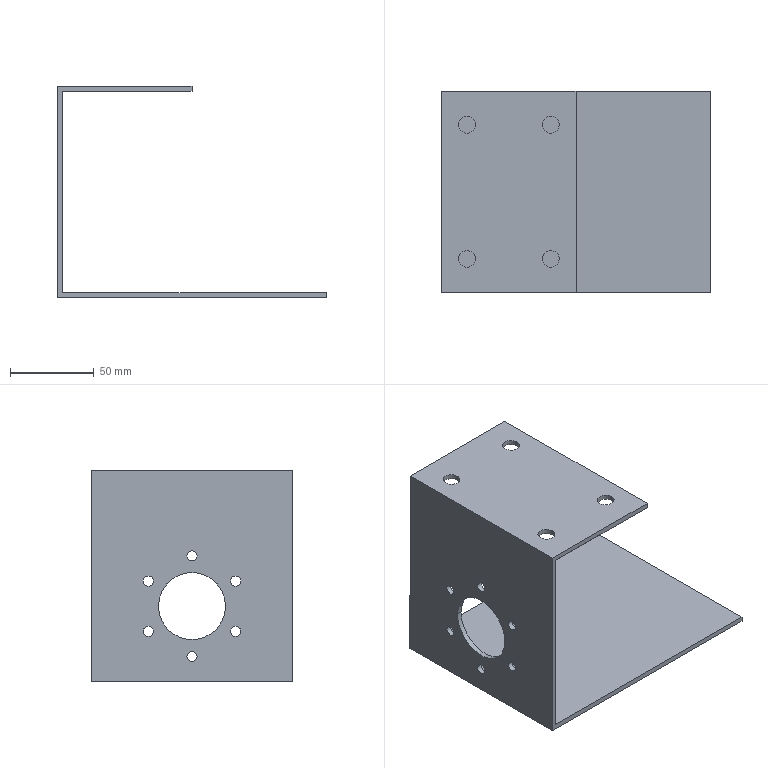Component | SolidWorks | MotorMount-1 | 1 solid | 32 faces | box 160 x 120 x 126 mm | volume 124379 mm3 | cylinder 22 | plane 10 | commonest cylinder face diameters 6 x12 10 x8 40 x2
STEP:
#1=CARTESIAN_POINT('',(-6.589,-12.89,16.22));
#2=VERTEX_POINT('',#1);
#3=CARTESIAN_POINT('',(-6.196,-12.89,16.22));
#4=VERTEX_POINT('',#3);
#5=CARTESIAN_POINT('',(-6.393,-12.89,16.22));
#6=DIRECTION('',(0.,-0.,1.));
#7=DIRECTION('',(1.,0.,0.));
#8=AXIS2_PLACEMENT_3D('',#5,#6,#7);
#9=CIRCLE('',#8,0.1969);
#10=EDGE_CURVE('',#2,#4,#9,.T.);
#11=ORIENTED_EDGE('',*,*,#10,.F.);
#12=CARTESIAN_POINT('',(-6.589,-12.89,16.339));
#13=VERTEX_POINT('',#12);
#14=CARTESIAN_POINT('',(-6.589,-12.89,16.22));
#15=DIRECTION('',(0.,-0.,1.));
#16=VECTOR('',#15,39.37);
#17=LINE('',#14,#16);
#18=EDGE_CURVE('',#2,#13,#17,.T.);
#19=ORIENTED_EDGE('',*,*,#18,.T.);
#20=CARTESIAN_POINT('',(-6.196,-12.89,16.339));
#21=VERTEX_POINT('',#20);
#22=CARTESIAN_POINT('',(-6.393,-12.89,16.339));
#23=DIRECTION('',(0.,-0.,1.));
#24=DIRECTION('',(1.,0.,0.));
#25=AXIS2_PLACEMENT_3D('',#22,#23,#24);
#26=CIRCLE('',#25,0.1969);
#27=EDGE_CURVE('',#13,#21,#26,.T.);
#28=ORIENTED_EDGE('',*,*,#27,.T.);
#29=CARTESIAN_POINT('',(-6.196,-12.89,16.22));
#30=DIRECTION('',(0.,-0.,1.));
#31=VECTOR('',#30,39.37);
#32=LINE('',#29,#31);
#33=EDGE_CURVE('',#4,#21,#32,.T.);
#34=ORIENTED_EDGE('',*,*,#33,.F.);
#35=EDGE_LOOP('',(#11,#19,#28,#34));
#36=FACE_OUTER_BOUND('',#35,.T.);
#37=CARTESIAN_POINT('',(-6.393,-12.89,16.22));
#38=DIRECTION('',(0.,-0.,1.));
#39=DIRECTION('',(1.,0.,0.));
#40=AXIS2_PLACEMENT_3D('',#37,#38,#39);
#41=CYLINDRICAL_SURFACE('',#40,0.1969);
#42=ADVANCED_FACE('',(#36),#41,.F.);
#43=CARTESIAN_POINT('',(-8.558,-16.04,16.22));
#44=VERTEX_POINT('',#43);
#45=CARTESIAN_POINT('',(-8.164,-16.04,16.22));
#46=VERTEX_POINT('',#45);
#47=CARTESIAN_POINT('',(-8.361,-16.04,16.22));
#48=DIRECTION('',(0.,-0.,1.));
#49=DIRECTION('',(1.,0.,0.));
#50=AXIS2_PLACEMENT_3D('',#47,#48,#49);
#51=CIRCLE('',#50,0.1969);
#52=EDGE_CURVE('',#44,#46,#51,.T.);
#53=ORIENTED_EDGE('',*,*,#52,.F.);
#54=CARTESIAN_POINT('',(-8.558,-16.04,16.339));
#55=VERTEX_POINT('',#54);
#56=CARTESIAN_POINT('',(-8.558,-16.04,16.22));
#57=DIRECTION('',(0.,-0.,1.));
#58=VECTOR('',#57,39.37);
#59=LINE('',#56,#58);
#60=EDGE_CURVE('',#44,#55,#59,.T.);
#61=ORIENTED_EDGE('',*,*,#60,.T.);
#62=CARTESIAN_POINT('',(-8.164,-16.04,16.339));
#63=VERTEX_POINT('',#62);
#64=CARTESIAN_POINT('',(-8.361,-16.04,16.339));
#65=DIRECTION('',(0.,-0.,1.));
#66=DIRECTION('',(1.,0.,0.));
#67=AXIS2_PLACEMENT_3D('',#64,#65,#66);
#68=CIRCLE('',#67,0.1969);
#69=EDGE_CURVE('',#55,#63,#68,.T.);
#70=ORIENTED_EDGE('',*,*,#69,.T.);
#71=CARTESIAN_POINT('',(-8.164,-16.04,16.22));
#72=DIRECTION('',(0.,-0.,1.));
#73=VECTOR('',#72,39.37);
#74=LINE('',#71,#73);
#75=EDGE_CURVE('',#46,#63,#74,.T.);
#76=ORIENTED_EDGE('',*,*,#75,.F.);
#77=EDGE_LOOP('',(#53,#61,#70,#76));
#78=FACE_OUTER_BOUND('',#77,.T.);
#79=CARTESIAN_POINT('',(-8.361,-16.04,16.22));
#80=DIRECTION('',(0.,-0.,1.));
#81=DIRECTION('',(1.,0.,0.));
#82=AXIS2_PLACEMENT_3D('',#79,#80,#81);
#83=CYLINDRICAL_SURFACE('',#82,0.1969);
#84=ADVANCED_FACE('',(#78),#83,.F.);
#85=CARTESIAN_POINT('',(-6.589,-16.04,16.22));
#86=VERTEX_POINT('',#85);
#87=CARTESIAN_POINT('',(-6.196,-16.04,16.22));
#88=VERTEX_POINT('',#87);
#89=CARTESIAN_POINT('',(-6.393,-16.04,16.22));
#90=DIRECTION('',(0.,-0.,1.));
#91=DIRECTION('',(1.,0.,0.));
#92=AXIS2_PLACEMENT_3D('',#89,#90,#91);
#93=CIRCLE('',#92,0.1969);
#94=EDGE_CURVE('',#86,#88,#93,.T.);
#95=ORIENTED_EDGE('',*,*,#94,.F.);
#96=CARTESIAN_POINT('',(-6.589,-16.04,16.339));
#97=VERTEX_POINT('',#96);
#98=CARTESIAN_POINT('',(-6.589,-16.04,16.22));
#99=DIRECTION('',(0.,-0.,1.));
#100=VECTOR('',#99,39.37);
#101=LINE('',#98,#100);
#102=EDGE_CURVE('',#86,#97,#101,.T.);
#103=ORIENTED_EDGE('',*,*,#102,.T.);
#104=CARTESIAN_POINT('',(-6.196,-16.04,16.339));
#105=VERTEX_POINT('',#104);
#106=CARTESIAN_POINT('',(-6.393,-16.04,16.339));
#107=DIRECTION('',(0.,-0.,1.));
#108=DIRECTION('',(1.,0.,0.));
#109=AXIS2_PLACEMENT_3D('',#106,#107,#108);
#110=CIRCLE('',#109,0.1969);
#111=EDGE_CURVE('',#97,#105,#110,.T.);
#112=ORIENTED_EDGE('',*,*,#111,.T.);
#113=CARTESIAN_POINT('',(-6.196,-16.04,16.22));
#114=DIRECTION('',(0.,-0.,1.));
#115=VECTOR('',#114,39.37);
#116=LINE('',#113,#115);
#117=EDGE_CURVE('',#88,#105,#116,.T.);
#118=ORIENTED_EDGE('',*,*,#117,.F.);
#119=EDGE_LOOP('',(#95,#103,#112,#118));
#120=FACE_OUTER_BOUND('',#119,.T.);
#121=CARTESIAN_POINT('',(-6.393,-16.04,16.22));
#122=DIRECTION('',(0.,-0.,1.));
#123=DIRECTION('',(1.,0.,0.));
#124=AXIS2_PLACEMENT_3D('',#121,#122,#123);
#125=CYLINDRICAL_SURFACE('',#124,0.1969);
#126=ADVANCED_FACE('',(#120),#125,.F.);
#127=CARTESIAN_POINT('',(-8.558,-12.89,16.22));
#128=VERTEX_POINT('',#127);
#129=CARTESIAN_POINT('',(-8.164,-12.89,16.22));
#130=VERTEX_POINT('',#129);
#131=CARTESIAN_POINT('',(-8.361,-12.89,16.22));
#132=DIRECTION('',(0.,-0.,1.));
#133=DIRECTION('',(1.,0.,0.));
#134=AXIS2_PLACEMENT_3D('',#131,#132,#133);
#135=CIRCLE('',#134,0.1969);
#136=EDGE_CURVE('',#128,#130,#135,.T.);
#137=ORIENTED_EDGE('',*,*,#136,.F.);
#138=CARTESIAN_POINT('',(-8.558,-12.89,16.339));
#139=VERTEX_POINT('',#138);
#140=CARTESIAN_POINT('',(-8.558,-12.89,16.22));
#141=DIRECTION('',(0.,-0.,1.));
#142=VECTOR('',#141,39.37);
#143=LINE('',#140,#142);
#144=EDGE_CURVE('',#128,#139,#143,.T.);
#145=ORIENTED_EDGE('',*,*,#144,.T.);
#146=CARTESIAN_POINT('',(-8.164,-12.89,16.339));
#147=VERTEX_POINT('',#146);
#148=CARTESIAN_POINT('',(-8.361,-12.89,16.339));
#149=DIRECTION('',(0.,-0.,1.));
#150=DIRECTION('',(1.,0.,0.));
#151=AXIS2_PLACEMENT_3D('',#148,#149,#150);
#152=CIRCLE('',#151,0.1969);
#153=EDGE_CURVE('',#139,#147,#152,.T.);
#154=ORIENTED_EDGE('',*,*,#153,.T.);
#155=CARTESIAN_POINT('',(-8.164,-12.89,16.22));
#156=DIRECTION('',(0.,-0.,1.));
#157=VECTOR('',#156,39.37);
#158=LINE('',#155,#157);
#159=EDGE_CURVE('',#130,#147,#158,.T.);
#160=ORIENTED_EDGE('',*,*,#159,.F.);
#161=EDGE_LOOP('',(#137,#145,#154,#160));
#162=FACE_OUTER_BOUND('',#161,.T.);
#163=CARTESIAN_POINT('',(-8.361,-12.89,16.22));
#164=DIRECTION('',(0.,-0.,1.));
#165=DIRECTION('',(1.,0.,0.));
#166=AXIS2_PLACEMENT_3D('',#163,#164,#165);
#167=CYLINDRICAL_SURFACE('',#166,0.1969);
#168=ADVANCED_FACE('',(#162),#167,.F.);
#169=CARTESIAN_POINT('',(-8.952,-13.677,13.15));
#170=VERTEX_POINT('',#169);
#171=CARTESIAN_POINT('',(-8.952,-15.252,13.15));
#172=VERTEX_POINT('',#171);
#173=CARTESIAN_POINT('',(-8.952,-14.465,13.15));
#174=DIRECTION('',(-1.,-0.,0.));
#175=DIRECTION('',(0.,-1.,0.));
#176=AXIS2_PLACEMENT_3D('',#173,#174,#175);
#177=CIRCLE('',#176,0.7874);
#178=EDGE_CURVE('',#170,#172,#177,.T.);
#179=ORIENTED_EDGE('',*,*,#178,.T.);
#180=CARTESIAN_POINT('',(-8.833,-15.252,13.15));
#181=VERTEX_POINT('',#180);
#182=CARTESIAN_POINT('',(-9.778,-15.252,13.15));
#183=DIRECTION('',(1.,0.,-0.));
#184=VECTOR('',#183,39.37);
#185=LINE('',#182,#184);
#186=EDGE_CURVE('',#172,#181,#185,.T.);
#187=ORIENTED_EDGE('',*,*,#186,.T.);
#188=CARTESIAN_POINT('',(-8.833,-13.677,13.15));
#189=VERTEX_POINT('',#188);
#190=CARTESIAN_POINT('',(-8.833,-14.465,13.15));
#191=DIRECTION('',(1.,0.,-0.));
#192=DIRECTION('',(0.,1.,0.));
#193=AXIS2_PLACEMENT_3D('',#190,#191,#192);
#194=CIRCLE('',#193,0.7874);
#195=EDGE_CURVE('',#181,#189,#194,.T.);
#196=ORIENTED_EDGE('',*,*,#195,.T.);
#197=CARTESIAN_POINT('',(-9.778,-13.677,13.15));
#198=DIRECTION('',(1.,0.,-0.));
#199=VECTOR('',#198,39.37);
#200=LINE('',#197,#199);
#201=EDGE_CURVE('',#170,#189,#200,.T.);
#202=ORIENTED_EDGE('',*,*,#201,.F.);
#203=EDGE_LOOP('',(#179,#187,#196,#202));
#204=FACE_OUTER_BOUND('',#203,.T.);
#205=CARTESIAN_POINT('',(-9.778,-14.465,13.15));
#206=DIRECTION('',(1.,0.,-0.));
#207=DIRECTION('',(0.,1.,0.));
#208=AXIS2_PLACEMENT_3D('',#205,#206,#207);
#209=CYLINDRICAL_SURFACE('',#208,0.7874);
#210=ADVANCED_FACE('',(#204),#209,.F.);
#211=CARTESIAN_POINT('',(-8.833,-14.347,14.331));
#212=VERTEX_POINT('',#211);
#213=CARTESIAN_POINT('',(-8.833,-14.583,14.331));
#214=VERTEX_POINT('',#213);
#215=CARTESIAN_POINT('',(-8.833,-14.465,14.331));
#216=DIRECTION('',(-1.,-0.,0.));
#217=DIRECTION('',(0.,-1.,0.));
#218=AXIS2_PLACEMENT_3D('',#215,#216,#217);
#219=CIRCLE('',#218,0.1181);
#220=EDGE_CURVE('',#212,#214,#219,.T.);
#221=ORIENTED_EDGE('',*,*,#220,.F.);
#222=CARTESIAN_POINT('',(-8.952,-14.347,14.331));
#223=VERTEX_POINT('',#222);
#224=CARTESIAN_POINT('',(-8.833,-14.347,14.331));
#225=DIRECTION('',(-1.,-0.,0.));
#226=VECTOR('',#225,39.37);
#227=LINE('',#224,#226);
#228=EDGE_CURVE('',#212,#223,#227,.T.);
#229=ORIENTED_EDGE('',*,*,#228,.T.);
#230=CARTESIAN_POINT('',(-8.952,-14.583,14.331));
#231=VERTEX_POINT('',#230);
#232=CARTESIAN_POINT('',(-8.952,-14.465,14.331));
#233=DIRECTION('',(-1.,-0.,0.));
#234=DIRECTION('',(0.,-1.,0.));
#235=AXIS2_PLACEMENT_3D('',#232,#233,#234);
#236=CIRCLE('',#235,0.1181);
#237=EDGE_CURVE('',#223,#231,#236,.T.);
#238=ORIENTED_EDGE('',*,*,#237,.T.);
#239=CARTESIAN_POINT('',(-8.833,-14.583,14.331));
#240=DIRECTION('',(-1.,-0.,0.));
#241=VECTOR('',#240,39.37);
#242=LINE('',#239,#241);
#243=EDGE_CURVE('',#214,#231,#242,.T.);
#244=ORIENTED_EDGE('',*,*,#243,.F.);
#245=EDGE_LOOP('',(#221,#229,#238,#244));
#246=FACE_OUTER_BOUND('',#245,.T.);
#247=CARTESIAN_POINT('',(-8.833,-14.465,14.331));
#248=DIRECTION('',(-1.,-0.,0.));
#249=DIRECTION('',(0.,-1.,0.));
#250=AXIS2_PLACEMENT_3D('',#247,#248,#249);
#251=CYLINDRICAL_SURFACE('',#250,0.1181);
#252=ADVANCED_FACE('',(#246),#251,.F.);
#253=CARTESIAN_POINT('',(-8.833,-13.324,13.74));
#254=VERTEX_POINT('',#253);
#255=CARTESIAN_POINT('',(-8.833,-13.56,13.74));
#256=VERTEX_POINT('',#255);
#257=CARTESIAN_POINT('',(-8.833,-13.442,13.74));
#258=DIRECTION('',(-1.,-0.,0.));
#259=DIRECTION('',(0.,-1.,0.));
#260=AXIS2_PLACEMENT_3D('',#257,#258,#259);
#261=CIRCLE('',#260,0.1181);
#262=EDGE_CURVE('',#254,#256,#261,.T.);
#263=ORIENTED_EDGE('',*,*,#262,.F.);
#264=CARTESIAN_POINT('',(-8.952,-13.324,13.74));
#265=VERTEX_POINT('',#264);
#266=CARTESIAN_POINT('',(-8.833,-13.324,13.74));
#267=DIRECTION('',(-1.,-0.,0.));
#268=VECTOR('',#267,39.37);
#269=LINE('',#266,#268);
#270=EDGE_CURVE('',#254,#265,#269,.T.);
#271=ORIENTED_EDGE('',*,*,#270,.T.);
#272=CARTESIAN_POINT('',(-8.952,-13.56,13.74));
#273=VERTEX_POINT('',#272);
#274=CARTESIAN_POINT('',(-8.952,-13.442,13.74));
#275=DIRECTION('',(-1.,-0.,0.));
#276=DIRECTION('',(0.,-1.,0.));
#277=AXIS2_PLACEMENT_3D('',#274,#275,#276);
#278=CIRCLE('',#277,0.1181);
#279=EDGE_CURVE('',#265,#273,#278,.T.);
#280=ORIENTED_EDGE('',*,*,#279,.T.);
#281=CARTESIAN_POINT('',(-8.833,-13.56,13.74));
#282=DIRECTION('',(-1.,-0.,0.));
#283=VECTOR('',#282,39.37);
#284=LINE('',#281,#283);
#285=EDGE_CURVE('',#256,#273,#284,.T.);
#286=ORIENTED_EDGE('',*,*,#285,.F.);
#287=EDGE_LOOP('',(#263,#271,#280,#286));
#288=FACE_OUTER_BOUND('',#287,.T.);
#289=CARTESIAN_POINT('',(-8.833,-13.442,13.74));
#290=DIRECTION('',(-1.,-0.,0.));
#291=DIRECTION('',(0.,-1.,0.));
#292=AXIS2_PLACEMENT_3D('',#289,#290,#291);
#293=CYLINDRICAL_SURFACE('',#292,0.1181);
#294=ADVANCED_FACE('',(#288),#293,.F.);
#295=CARTESIAN_POINT('',(-8.833,-13.324,12.559));
#296=VERTEX_POINT('',#295);
#297=CARTESIAN_POINT('',(-8.833,-13.56,12.559));
#298=VERTEX_POINT('',#297);
#299=CARTESIAN_POINT('',(-8.833,-13.442,12.559));
#300=DIRECTION('',(-1.,-0.,0.));
#301=DIRECTION('',(0.,-1.,0.));
#302=AXIS2_PLACEMENT_3D('',#299,#300,#301);
#303=CIRCLE('',#302,0.1181);
#304=EDGE_CURVE('',#296,#298,#303,.T.);
#305=ORIENTED_EDGE('',*,*,#304,.F.);
#306=CARTESIAN_POINT('',(-8.952,-13.324,12.559));
#307=VERTEX_POINT('',#306);
#308=CARTESIAN_POINT('',(-8.833,-13.324,12.559));
#309=DIRECTION('',(-1.,-0.,0.));
#310=VECTOR('',#309,39.37);
#311=LINE('',#308,#310);
#312=EDGE_CURVE('',#296,#307,#311,.T.);
#313=ORIENTED_EDGE('',*,*,#312,.T.);
#314=CARTESIAN_POINT('',(-8.952,-13.56,12.559));
#315=VERTEX_POINT('',#314);
#316=CARTESIAN_POINT('',(-8.952,-13.442,12.559));
#317=DIRECTION('',(-1.,-0.,0.));
#318=DIRECTION('',(0.,-1.,0.));
#319=AXIS2_PLACEMENT_3D('',#316,#317,#318);
#320=CIRCLE('',#319,0.1181);
#321=EDGE_CURVE('',#307,#315,#320,.T.);
#322=ORIENTED_EDGE('',*,*,#321,.T.);
#323=CARTESIAN_POINT('',(-8.833,-13.56,12.559));
#324=DIRECTION('',(-1.,-0.,0.));
#325=VECTOR('',#324,39.37);
#326=LINE('',#323,#325);
#327=EDGE_CURVE('',#298,#315,#326,.T.);
#328=ORIENTED_EDGE('',*,*,#327,.F.);
#329=EDGE_LOOP('',(#305,#313,#322,#328));
#330=FACE_OUTER_BOUND('',#329,.T.);
#331=CARTESIAN_POINT('',(-8.833,-13.442,12.559));
#332=DIRECTION('',(-1.,-0.,0.));
#333=DIRECTION('',(0.,-1.,0.));
#334=AXIS2_PLACEMENT_3D('',#331,#332,#333);
#335=CYLINDRICAL_SURFACE('',#334,0.1181);
#336=ADVANCED_FACE('',(#330),#335,.F.);
#337=CARTESIAN_POINT('',(-8.833,-14.347,11.969));
#338=VERTEX_POINT('',#337);
#339=CARTESIAN_POINT('',(-8.833,-14.583,11.969));
#340=VERTEX_POINT('',#339);
#341=CARTESIAN_POINT('',(-8.833,-14.465,11.969));
#342=DIRECTION('',(-1.,-0.,0.));
#343=DIRECTION('',(0.,-1.,0.));
#344=AXIS2_PLACEMENT_3D('',#341,#342,#343);
#345=CIRCLE('',#344,0.1181);
#346=EDGE_CURVE('',#338,#340,#345,.T.);
#347=ORIENTED_EDGE('',*,*,#346,.F.);
#348=CARTESIAN_POINT('',(-8.952,-14.347,11.969));
#349=VERTEX_POINT('',#348);
#350=CARTESIAN_POINT('',(-8.833,-14.347,11.969));
#351=DIRECTION('',(-1.,-0.,0.));
#352=VECTOR('',#351,39.37);
#353=LINE('',#350,#352);
#354=EDGE_CURVE('',#338,#349,#353,.T.);
#355=ORIENTED_EDGE('',*,*,#354,.T.);
#356=CARTESIAN_POINT('',(-8.952,-14.583,11.969));
#357=VERTEX_POINT('',#356);
#358=CARTESIAN_POINT('',(-8.952,-14.465,11.969));
#359=DIRECTION('',(-1.,-0.,0.));
#360=DIRECTION('',(0.,-1.,0.));
#361=AXIS2_PLACEMENT_3D('',#358,#359,#360);
#362=CIRCLE('',#361,0.1181);
#363=EDGE_CURVE('',#349,#357,#362,.T.);
#364=ORIENTED_EDGE('',*,*,#363,.T.);
#365=CARTESIAN_POINT('',(-8.833,-14.583,11.969));
#366=DIRECTION('',(-1.,-0.,0.));
#367=VECTOR('',#366,39.37);
#368=LINE('',#365,#367);
#369=EDGE_CURVE('',#340,#357,#368,.T.);
#370=ORIENTED_EDGE('',*,*,#369,.F.);
#371=EDGE_LOOP('',(#347,#355,#364,#370));
#372=FACE_OUTER_BOUND('',#371,.T.);
#373=CARTESIAN_POINT('',(-8.833,-14.465,11.969));
#374=DIRECTION('',(-1.,-0.,0.));
#375=DIRECTION('',(0.,-1.,0.));
#376=AXIS2_PLACEMENT_3D('',#373,#374,#375);
#377=CYLINDRICAL_SURFACE('',#376,0.1181);
#378=ADVANCED_FACE('',(#372),#377,.F.);
#379=CARTESIAN_POINT('',(-8.833,-15.37,12.559));
#380=VERTEX_POINT('',#379);
#381=CARTESIAN_POINT('',(-8.833,-15.606,12.559));
#382=VERTEX_POINT('',#381);
#383=CARTESIAN_POINT('',(-8.833,-15.488,12.559));
#384=DIRECTION('',(-1.,-0.,0.));
#385=DIRECTION('',(0.,-1.,0.));
#386=AXIS2_PLACEMENT_3D('',#383,#384,#385);
#387=CIRCLE('',#386,0.1181);
#388=EDGE_CURVE('',#380,#382,#387,.T.);
#389=ORIENTED_EDGE('',*,*,#388,.F.);
#390=CARTESIAN_POINT('',(-8.952,-15.37,12.559));
#391=VERTEX_POINT('',#390);
#392=CARTESIAN_POINT('',(-8.833,-15.37,12.559));
#393=DIRECTION('',(-1.,-0.,0.));
#394=VECTOR('',#393,39.37);
#395=LINE('',#392,#394);
#396=EDGE_CURVE('',#380,#391,#395,.T.);
#397=ORIENTED_EDGE('',*,*,#396,.T.);
#398=CARTESIAN_POINT('',(-8.952,-15.606,12.559));
#399=VERTEX_POINT('',#398);
#400=CARTESIAN_POINT('',(-8.952,-15.488,12.559));
#401=DIRECTION('',(-1.,-0.,0.));
#402=DIRECTION('',(0.,-1.,0.));
#403=AXIS2_PLACEMENT_3D('',#400,#401,#402);
#404=CIRCLE('',#403,0.1181);
#405=EDGE_CURVE('',#391,#399,#404,.T.);
#406=ORIENTED_EDGE('',*,*,#405,.T.);
#407=CARTESIAN_POINT('',(-8.833,-15.606,12.559));
#408=DIRECTION('',(-1.,-0.,0.));
#409=VECTOR('',#408,39.37);
#410=LINE('',#407,#409);
#411=EDGE_CURVE('',#382,#399,#410,.T.);
#412=ORIENTED_EDGE('',*,*,#411,.F.);
#413=EDGE_LOOP('',(#389,#397,#406,#412));
#414=FACE_OUTER_BOUND('',#413,.T.);
#415=CARTESIAN_POINT('',(-8.833,-15.488,12.559));
#416=DIRECTION('',(-1.,-0.,0.));
#417=DIRECTION('',(0.,-1.,0.));
#418=AXIS2_PLACEMENT_3D('',#415,#416,#417);
#419=CYLINDRICAL_SURFACE('',#418,0.1181);
#420=ADVANCED_FACE('',(#414),#419,.F.);
#421=CARTESIAN_POINT('',(-8.833,-15.37,13.74));
#422=VERTEX_POINT('',#421);
#423=CARTESIAN_POINT('',(-8.833,-15.606,13.74));
#424=VERTEX_POINT('',#423);
#425=CARTESIAN_POINT('',(-8.833,-15.488,13.74));
#426=DIRECTION('',(-1.,-0.,0.));
#427=DIRECTION('',(0.,-1.,0.));
#428=AXIS2_PLACEMENT_3D('',#425,#426,#427);
#429=CIRCLE('',#428,0.1181);
#430=EDGE_CURVE('',#422,#424,#429,.T.);
#431=ORIENTED_EDGE('',*,*,#430,.F.);
#432=CARTESIAN_POINT('',(-8.952,-15.37,13.74));
#433=VERTEX_POINT('',#432);
#434=CARTESIAN_POINT('',(-8.833,-15.37,13.74));
#435=DIRECTION('',(-1.,-0.,0.));
#436=VECTOR('',#435,39.37);
#437=LINE('',#434,#436);
#438=EDGE_CURVE('',#422,#433,#437,.T.);
#439=ORIENTED_EDGE('',*,*,#438,.T.);
#440=CARTESIAN_POINT('',(-8.952,-15.606,13.74));
#441=VERTEX_POINT('',#440);
#442=CARTESIAN_POINT('',(-8.952,-15.488,13.74));
#443=DIRECTION('',(-1.,-0.,0.));
#444=DIRECTION('',(0.,-1.,0.));
#445=AXIS2_PLACEMENT_3D('',#442,#443,#444);
#446=CIRCLE('',#445,0.1181);
#447=EDGE_CURVE('',#433,#441,#446,.T.);
#448=ORIENTED_EDGE('',*,*,#447,.T.);
#449=CARTESIAN_POINT('',(-8.833,-15.606,13.74));
#450=DIRECTION('',(-1.,-0.,0.));
#451=VECTOR('',#450,39.37);
#452=LINE('',#449,#451);
#453=EDGE_CURVE('',#424,#441,#452,.T.);
#454=ORIENTED_EDGE('',*,*,#453,.F.);
#455=EDGE_LOOP('',(#431,#439,#448,#454));
#456=FACE_OUTER_BOUND('',#455,.T.);
#457=CARTESIAN_POINT('',(-8.833,-15.488,13.74));
#458=DIRECTION('',(-1.,-0.,0.));
#459=DIRECTION('',(0.,-1.,0.));
#460=AXIS2_PLACEMENT_3D('',#457,#458,#459);
#461=CYLINDRICAL_SURFACE('',#460,0.1181);
#462=ADVANCED_FACE('',(#456),#461,.F.);
#463=CARTESIAN_POINT('',(-8.952,-12.103,11.378));
#464=VERTEX_POINT('',#463);
#465=CARTESIAN_POINT('',(-8.952,-12.103,16.339));
#466=VERTEX_POINT('',#465);
#467=CARTESIAN_POINT('',(-8.952,-12.103,11.496));
#468=DIRECTION('',(0.,-0.,1.));
#469=VECTOR('',#468,39.37);
#470=LINE('',#467,#469);
#471=EDGE_CURVE('',#464,#466,#470,.T.);
#472=ORIENTED_EDGE('',*,*,#471,.T.);
#473=CARTESIAN_POINT('',(-5.802,-12.103,16.339));
#474=VERTEX_POINT('',#473);
#475=CARTESIAN_POINT('',(-8.952,-12.103,16.339));
#476=DIRECTION('',(-1.,-0.,0.));
#477=VECTOR('',#476,39.37);
#478=LINE('',#475,#477);
#479=EDGE_CURVE('',#474,#466,#478,.T.);
#480=ORIENTED_EDGE('',*,*,#479,.F.);
#481=CARTESIAN_POINT('',(-5.802,-12.103,16.22));
#482=VERTEX_POINT('',#481);
#483=CARTESIAN_POINT('',(-5.802,-12.103,16.339));
#484=DIRECTION('',(-0.,0.,-1.));
#485=VECTOR('',#484,39.37);
#486=LINE('',#483,#485);
#487=EDGE_CURVE('',#474,#482,#486,.T.);
#488=ORIENTED_EDGE('',*,*,#487,.T.);
#489=CARTESIAN_POINT('',(-8.833,-12.103,16.22));
#490=VERTEX_POINT('',#489);
#491=CARTESIAN_POINT('',(-8.952,-12.103,16.22));
#492=DIRECTION('',(-1.,-0.,0.));
#493=VECTOR('',#492,39.37);
#494=LINE('',#491,#493);
#495=EDGE_CURVE('',#482,#490,#494,.T.);
#496=ORIENTED_EDGE('',*,*,#495,.T.);
#497=CARTESIAN_POINT('',(-8.833,-12.103,11.496));
#498=VERTEX_POINT('',#497);
#499=CARTESIAN_POINT('',(-8.833,-12.103,11.496));
#500=DIRECTION('',(0.,-0.,1.));
#501=VECTOR('',#500,39.37);
#502=LINE('',#499,#501);
#503=EDGE_CURVE('',#498,#490,#502,.T.);
#504=ORIENTED_EDGE('',*,*,#503,.F.);
#505=CARTESIAN_POINT('',(-2.652,-12.103,11.496));
#506=VERTEX_POINT('',#505);
#507=CARTESIAN_POINT('',(-8.952,-12.103,11.496));
#508=DIRECTION('',(1.,0.,-0.));
#509=VECTOR('',#508,39.37);
#510=LINE('',#507,#509);
#511=EDGE_CURVE('',#498,#506,#510,.T.);
#512=ORIENTED_EDGE('',*,*,#511,.T.);
#513=CARTESIAN_POINT('',(-2.652,-12.103,11.378));
#514=VERTEX_POINT('',#513);
#515=CARTESIAN_POINT('',(-2.652,-12.103,11.378));
#516=DIRECTION('',(0.,-0.,1.));
#517=VECTOR('',#516,39.37);
#518=LINE('',#515,#517);
#519=EDGE_CURVE('',#514,#506,#518,.T.);
#520=ORIENTED_EDGE('',*,*,#519,.F.);
#521=CARTESIAN_POINT('',(-8.952,-12.103,11.378));
#522=DIRECTION('',(1.,0.,-0.));
#523=VECTOR('',#522,39.37);
#524=LINE('',#521,#523);
#525=EDGE_CURVE('',#464,#514,#524,.T.);
#526=ORIENTED_EDGE('',*,*,#525,.F.);
#527=EDGE_LOOP('',(#472,#480,#488,#496,#504,#512,#520,#526));
#528=FACE_OUTER_BOUND('',#527,.T.);
#529=CARTESIAN_POINT('',(-8.833,-12.103,11.496));
#530=DIRECTION('',(0.,-1.,-0.));
#531=DIRECTION('',(1.,0.,-0.));
#532=AXIS2_PLACEMENT_3D('',#529,#530,#531);
#533=PLANE('',#532);
#534=ADVANCED_FACE('',(#528),#533,.F.);
#535=CARTESIAN_POINT('',(-8.952,-16.827,16.339));
#536=VERTEX_POINT('',#535);
#537=CARTESIAN_POINT('',(-8.952,-16.827,11.378));
#538=VERTEX_POINT('',#537);
#539=CARTESIAN_POINT('',(-8.952,-16.827,11.496));
#540=DIRECTION('',(-0.,0.,-1.));
#541=VECTOR('',#540,39.37);
#542=LINE('',#539,#541);
#543=EDGE_CURVE('',#536,#538,#542,.T.);
#544=ORIENTED_EDGE('',*,*,#543,.T.);
#545=CARTESIAN_POINT('',(-2.652,-16.827,11.378));
#546=VERTEX_POINT('',#545);
#547=CARTESIAN_POINT('',(-2.652,-16.827,11.378));
#548=DIRECTION('',(-1.,0.,0.));
#549=VECTOR('',#548,39.37);
#550=LINE('',#547,#549);
#551=EDGE_CURVE('',#546,#538,#550,.T.);
#552=ORIENTED_EDGE('',*,*,#551,.F.);
#553=CARTESIAN_POINT('',(-2.652,-16.827,11.496));
#554=VERTEX_POINT('',#553);
#555=CARTESIAN_POINT('',(-2.652,-16.827,11.378));
#556=DIRECTION('',(0.,-0.,1.));
#557=VECTOR('',#556,39.37);
#558=LINE('',#555,#557);
#559=EDGE_CURVE('',#546,#554,#558,.T.);
#560=ORIENTED_EDGE('',*,*,#559,.T.);
#561=CARTESIAN_POINT('',(-8.833,-16.827,11.496));
#562=VERTEX_POINT('',#561);
#563=CARTESIAN_POINT('',(-2.652,-16.827,11.496));
#564=DIRECTION('',(-1.,0.,0.));
#565=VECTOR('',#564,39.37);
#566=LINE('',#563,#565);
#567=EDGE_CURVE('',#554,#562,#566,.T.);
#568=ORIENTED_EDGE('',*,*,#567,.T.);
#569=CARTESIAN_POINT('',(-8.833,-16.827,16.22));
#570=VERTEX_POINT('',#569);
#571=CARTESIAN_POINT('',(-8.833,-16.827,11.496));
#572=DIRECTION('',(-0.,0.,-1.));
#573=VECTOR('',#572,39.37);
#574=LINE('',#571,#573);
#575=EDGE_CURVE('',#570,#562,#574,.T.);
#576=ORIENTED_EDGE('',*,*,#575,.F.);
#577=CARTESIAN_POINT('',(-5.802,-16.827,16.22));
#578=VERTEX_POINT('',#577);
#579=CARTESIAN_POINT('',(-8.952,-16.827,16.22));
#580=DIRECTION('',(1.,0.,-0.));
#581=VECTOR('',#580,39.37);
#582=LINE('',#579,#581);
#583=EDGE_CURVE('',#570,#578,#582,.T.);
#584=ORIENTED_EDGE('',*,*,#583,.T.);
#585=CARTESIAN_POINT('',(-5.802,-16.827,16.339));
#586=VERTEX_POINT('',#585);
#587=CARTESIAN_POINT('',(-5.802,-16.827,16.339));
#588=DIRECTION('',(-0.,0.,-1.));
#589=VECTOR('',#588,39.37);
#590=LINE('',#587,#589);
#591=EDGE_CURVE('',#586,#578,#590,.T.);
#592=ORIENTED_EDGE('',*,*,#591,.F.);
#593=CARTESIAN_POINT('',(-8.952,-16.827,16.339));
#594=DIRECTION('',(1.,0.,-0.));
#595=VECTOR('',#594,39.37);
#596=LINE('',#593,#595);
#597=EDGE_CURVE('',#536,#586,#596,.T.);
#598=ORIENTED_EDGE('',*,*,#597,.F.);
#599=EDGE_LOOP('',(#544,#552,#560,#568,#576,#584,#592,#598));
#600=FACE_OUTER_BOUND('',#599,.T.);
#601=CARTESIAN_POINT('',(-8.833,-16.827,11.496));
#602=DIRECTION('',(-0.,1.,0.));
#603=DIRECTION('',(-1.,-0.,0.));
#604=AXIS2_PLACEMENT_3D('',#601,#602,#603);
#605=PLANE('',#604);
#606=ADVANCED_FACE('',(#600),#605,.F.);
#607=CARTESIAN_POINT('',(-8.833,-14.465,13.15));
#608=DIRECTION('',(1.,0.,-0.));
#609=DIRECTION('',(0.,1.,0.));
#610=AXIS2_PLACEMENT_3D('',#607,#608,#609);
#611=CIRCLE('',#610,0.7874);
#612=EDGE_CURVE('',#189,#181,#611,.T.);
#613=ORIENTED_EDGE('',*,*,#612,.F.);
#614=ORIENTED_EDGE('',*,*,#195,.F.);
#615=EDGE_LOOP('',(#613,#614));
#616=FACE_BOUND('',#615,.T.);
#617=CARTESIAN_POINT('',(-8.833,-14.465,14.331));
#618=DIRECTION('',(-1.,-0.,0.));
#619=DIRECTION('',(0.,-1.,0.));
#620=AXIS2_PLACEMENT_3D('',#617,#618,#619);
#621=CIRCLE('',#620,0.1181);
#622=EDGE_CURVE('',#214,#212,#621,.T.);
#623=ORIENTED_EDGE('',*,*,#622,.T.);
#624=ORIENTED_EDGE('',*,*,#220,.T.);
#625=EDGE_LOOP('',(#623,#624));
#626=FACE_BOUND('',#625,.T.);
#627=CARTESIAN_POINT('',(-8.833,-13.442,13.74));
#628=DIRECTION('',(-1.,-0.,0.));
#629=DIRECTION('',(0.,-1.,0.));
#630=AXIS2_PLACEMENT_3D('',#627,#628,#629);
#631=CIRCLE('',#630,0.1181);
#632=EDGE_CURVE('',#256,#254,#631,.T.);
#633=ORIENTED_EDGE('',*,*,#632,.T.);
#634=ORIENTED_EDGE('',*,*,#262,.T.);
#635=EDGE_LOOP('',(#633,#634));
#636=FACE_BOUND('',#635,.T.);
#637=CARTESIAN_POINT('',(-8.833,-13.442,12.559));
#638=DIRECTION('',(-1.,-0.,0.));
#639=DIRECTION('',(0.,-1.,0.));
#640=AXIS2_PLACEMENT_3D('',#637,#638,#639);
#641=CIRCLE('',#640,0.1181);
#642=EDGE_CURVE('',#298,#296,#641,.T.);
#643=ORIENTED_EDGE('',*,*,#642,.T.);
#644=ORIENTED_EDGE('',*,*,#304,.T.);
#645=EDGE_LOOP('',(#643,#644));
#646=FACE_BOUND('',#645,.T.);
#647=CARTESIAN_POINT('',(-8.833,-14.465,11.969));
#648=DIRECTION('',(-1.,-0.,0.));
#649=DIRECTION('',(0.,-1.,0.));
#650=AXIS2_PLACEMENT_3D('',#647,#648,#649);
#651=CIRCLE('',#650,0.1181);
#652=EDGE_CURVE('',#340,#338,#651,.T.);
#653=ORIENTED_EDGE('',*,*,#652,.T.);
#654=ORIENTED_EDGE('',*,*,#346,.T.);
#655=EDGE_LOOP('',(#653,#654));
#656=FACE_BOUND('',#655,.T.);
#657=CARTESIAN_POINT('',(-8.833,-15.488,12.559));
#658=DIRECTION('',(-1.,-0.,0.));
#659=DIRECTION('',(0.,-1.,0.));
#660=AXIS2_PLACEMENT_3D('',#657,#658,#659);
#661=CIRCLE('',#660,0.1181);
#662=EDGE_CURVE('',#382,#380,#661,.T.);
#663=ORIENTED_EDGE('',*,*,#662,.T.);
#664=ORIENTED_EDGE('',*,*,#388,.T.);
#665=EDGE_LOOP('',(#663,#664));
#666=FACE_BOUND('',#665,.T.);
#667=CARTESIAN_POINT('',(-8.833,-15.488,13.74));
#668=DIRECTION('',(-1.,-0.,0.));
#669=DIRECTION('',(0.,-1.,0.));
#670=AXIS2_PLACEMENT_3D('',#667,#668,#669);
#671=CIRCLE('',#670,0.1181);
#672=EDGE_CURVE('',#424,#422,#671,.T.);
#673=ORIENTED_EDGE('',*,*,#672,.T.);
#674=ORIENTED_EDGE('',*,*,#430,.T.);
#675=EDGE_LOOP('',(#673,#674));
#676=FACE_BOUND('',#675,.T.);
#677=ORIENTED_EDGE('',*,*,#503,.T.);
#678=CARTESIAN_POINT('',(-8.833,-16.827,16.22));
#679=DIRECTION('',(0.,-1.,-0.));
#680=VECTOR('',#679,39.37);
#681=LINE('',#678,#680);
#682=EDGE_CURVE('',#490,#570,#681,.T.);
#683=ORIENTED_EDGE('',*,*,#682,.T.);
#684=ORIENTED_EDGE('',*,*,#575,.T.);
#685=CARTESIAN_POINT('',(-8.833,-16.827,11.496));
#686=DIRECTION('',(-0.,1.,0.));
#687=VECTOR('',#686,39.37);
#688=LINE('',#685,#687);
#689=EDGE_CURVE('',#562,#498,#688,.T.);
#690=ORIENTED_EDGE('',*,*,#689,.T.);
#691=EDGE_LOOP('',(#677,#683,#684,#690));
#692=FACE_OUTER_BOUND('',#691,.T.);
#693=CARTESIAN_POINT('',(-8.833,-14.465,13.15));
#694=DIRECTION('',(-1.,-0.,0.));
#695=DIRECTION('',(0.,-1.,-0.));
#696=AXIS2_PLACEMENT_3D('',#693,#694,#695);
#697=PLANE('',#696);
#698=ADVANCED_FACE('',(#616,#626,#636,#646,#656,#666,#676,#692),#697,.F.);
#699=ORIENTED_EDGE('',*,*,#178,.F.);
#700=CARTESIAN_POINT('',(-8.952,-14.465,13.15));
#701=DIRECTION('',(-1.,-0.,0.));
#702=DIRECTION('',(0.,-1.,0.));
#703=AXIS2_PLACEMENT_3D('',#700,#701,#702);
#704=CIRCLE('',#703,0.7874);
#705=EDGE_CURVE('',#172,#170,#704,.T.);
#706=ORIENTED_EDGE('',*,*,#705,.F.);
#707=EDGE_LOOP('',(#699,#706));
#708=FACE_BOUND('',#707,.T.);
#709=CARTESIAN_POINT('',(-8.952,-14.465,14.331));
#710=DIRECTION('',(-1.,-0.,0.));
#711=DIRECTION('',(0.,-1.,0.));
#712=AXIS2_PLACEMENT_3D('',#709,#710,#711);
#713=CIRCLE('',#712,0.1181);
#714=EDGE_CURVE('',#231,#223,#713,.T.);
#715=ORIENTED_EDGE('',*,*,#714,.F.);
#716=ORIENTED_EDGE('',*,*,#237,.F.);
#717=EDGE_LOOP('',(#715,#716));
#718=FACE_BOUND('',#717,.T.);
#719=CARTESIAN_POINT('',(-8.952,-13.442,13.74));
#720=DIRECTION('',(-1.,-0.,0.));
#721=DIRECTION('',(0.,-1.,0.));
#722=AXIS2_PLACEMENT_3D('',#719,#720,#721);
#723=CIRCLE('',#722,0.1181);
#724=EDGE_CURVE('',#273,#265,#723,.T.);
#725=ORIENTED_EDGE('',*,*,#724,.F.);
#726=ORIENTED_EDGE('',*,*,#279,.F.);
#727=EDGE_LOOP('',(#725,#726));
#728=FACE_BOUND('',#727,.T.);
#729=CARTESIAN_POINT('',(-8.952,-13.442,12.559));
#730=DIRECTION('',(-1.,-0.,0.));
#731=DIRECTION('',(0.,-1.,0.));
#732=AXIS2_PLACEMENT_3D('',#729,#730,#731);
#733=CIRCLE('',#732,0.1181);
#734=EDGE_CURVE('',#315,#307,#733,.T.);
#735=ORIENTED_EDGE('',*,*,#734,.F.);
#736=ORIENTED_EDGE('',*,*,#321,.F.);
#737=EDGE_LOOP('',(#735,#736));
#738=FACE_BOUND('',#737,.T.);
#739=CARTESIAN_POINT('',(-8.952,-14.465,11.969));
#740=DIRECTION('',(-1.,-0.,0.));
#741=DIRECTION('',(0.,-1.,0.));
#742=AXIS2_PLACEMENT_3D('',#739,#740,#741);
#743=CIRCLE('',#742,0.1181);
#744=EDGE_CURVE('',#357,#349,#743,.T.);
#745=ORIENTED_EDGE('',*,*,#744,.F.);
#746=ORIENTED_EDGE('',*,*,#363,.F.);
#747=EDGE_LOOP('',(#745,#746));
#748=FACE_BOUND('',#747,.T.);
#749=CARTESIAN_POINT('',(-8.952,-15.488,12.559));
#750=DIRECTION('',(-1.,-0.,0.));
#751=DIRECTION('',(0.,-1.,0.));
#752=AXIS2_PLACEMENT_3D('',#749,#750,#751);
#753=CIRCLE('',#752,0.1181);
#754=EDGE_CURVE('',#399,#391,#753,.T.);
#755=ORIENTED_EDGE('',*,*,#754,.F.);
#756=ORIENTED_EDGE('',*,*,#405,.F.);
#757=EDGE_LOOP('',(#755,#756));
#758=FACE_BOUND('',#757,.T.);
#759=CARTESIAN_POINT('',(-8.952,-15.488,13.74));
#760=DIRECTION('',(-1.,-0.,0.));
#761=DIRECTION('',(0.,-1.,0.));
#762=AXIS2_PLACEMENT_3D('',#759,#760,#761);
#763=CIRCLE('',#762,0.1181);
#764=EDGE_CURVE('',#441,#433,#763,.T.);
#765=ORIENTED_EDGE('',*,*,#764,.F.);
#766=ORIENTED_EDGE('',*,*,#447,.F.);
#767=EDGE_LOOP('',(#765,#766));
#768=FACE_BOUND('',#767,.T.);
#769=ORIENTED_EDGE('',*,*,#471,.F.);
#770=CARTESIAN_POINT('',(-8.952,-16.827,11.378));
#771=DIRECTION('',(-0.,1.,0.));
#772=VECTOR('',#771,39.37);
#773=LINE('',#770,#772);
#774=EDGE_CURVE('',#538,#464,#773,.T.);
#775=ORIENTED_EDGE('',*,*,#774,.F.);
#776=ORIENTED_EDGE('',*,*,#543,.F.);
#777=CARTESIAN_POINT('',(-8.952,-16.827,16.339));
#778=DIRECTION('',(0.,-1.,-0.));
#779=VECTOR('',#778,39.37);
#780=LINE('',#777,#779);
#781=EDGE_CURVE('',#466,#536,#780,.T.);
#782=ORIENTED_EDGE('',*,*,#781,.F.);
#783=EDGE_LOOP('',(#769,#775,#776,#782));
#784=FACE_OUTER_BOUND('',#783,.T.);
#785=CARTESIAN_POINT('',(-8.952,-14.465,13.15));
#786=DIRECTION('',(-1.,-0.,0.));
#787=DIRECTION('',(0.,-1.,-0.));
#788=AXIS2_PLACEMENT_3D('',#785,#786,#787);
#789=PLANE('',#788);
#790=ADVANCED_FACE('',(#708,#718,#728,#738,#748,#758,#768,#784),#789,.T.);
#791=CARTESIAN_POINT('',(-2.652,-12.103,11.496));
#792=DIRECTION('',(0.,-1.,-0.));
#793=VECTOR('',#792,39.37);
#794=LINE('',#791,#793);
#795=EDGE_CURVE('',#506,#554,#794,.T.);
#796=ORIENTED_EDGE('',*,*,#795,.T.);
#797=ORIENTED_EDGE('',*,*,#559,.F.);
#798=CARTESIAN_POINT('',(-2.652,-12.103,11.378));
#799=DIRECTION('',(0.,-1.,-0.));
#800=VECTOR('',#799,39.37);
#801=LINE('',#798,#800);
#802=EDGE_CURVE('',#514,#546,#801,.T.);
#803=ORIENTED_EDGE('',*,*,#802,.F.);
#804=ORIENTED_EDGE('',*,*,#519,.T.);
#805=EDGE_LOOP('',(#796,#797,#803,#804));
#806=FACE_OUTER_BOUND('',#805,.T.);
#807=CARTESIAN_POINT('',(-2.652,-12.103,11.378));
#808=DIRECTION('',(-1.,-0.,0.));
#809=DIRECTION('',(0.,-1.,-0.));
#810=AXIS2_PLACEMENT_3D('',#807,#808,#809);
#811=PLANE('',#810);
#812=ADVANCED_FACE('',(#806),#811,.F.);
#813=ORIENTED_EDGE('',*,*,#551,.T.);
#814=ORIENTED_EDGE('',*,*,#774,.T.);
#815=ORIENTED_EDGE('',*,*,#525,.T.);
#816=ORIENTED_EDGE('',*,*,#802,.T.);
#817=EDGE_LOOP('',(#813,#814,#815,#816));
#818=FACE_OUTER_BOUND('',#817,.T.);
#819=CARTESIAN_POINT('',(-8.952,-14.465,11.378));
#820=DIRECTION('',(-0.,0.,-1.));
#821=DIRECTION('',(-1.,-0.,0.));
#822=AXIS2_PLACEMENT_3D('',#819,#820,#821);
#823=PLANE('',#822);
#824=ADVANCED_FACE('',(#818),#823,.T.);
#825=ORIENTED_EDGE('',*,*,#689,.F.);
#826=ORIENTED_EDGE('',*,*,#567,.F.);
#827=ORIENTED_EDGE('',*,*,#795,.F.);
#828=ORIENTED_EDGE('',*,*,#511,.F.);
#829=EDGE_LOOP('',(#825,#826,#827,#828));
#830=FACE_OUTER_BOUND('',#829,.T.);
#831=CARTESIAN_POINT('',(-8.952,-14.465,11.496));
#832=DIRECTION('',(-0.,0.,-1.));
#833=DIRECTION('',(-1.,-0.,0.));
#834=AXIS2_PLACEMENT_3D('',#831,#832,#833);
#835=PLANE('',#834);
#836=ADVANCED_FACE('',(#830),#835,.F.);
#837=ORIENTED_EDGE('',*,*,#438,.F.);
#838=ORIENTED_EDGE('',*,*,#672,.F.);
#839=ORIENTED_EDGE('',*,*,#453,.T.);
#840=ORIENTED_EDGE('',*,*,#764,.T.);
#841=EDGE_LOOP('',(#837,#838,#839,#840));
#842=FACE_OUTER_BOUND('',#841,.T.);
#843=CARTESIAN_POINT('',(-8.833,-15.488,13.74));
#844=DIRECTION('',(-1.,-0.,0.));
#845=DIRECTION('',(0.,-1.,0.));
#846=AXIS2_PLACEMENT_3D('',#843,#844,#845);
#847=CYLINDRICAL_SURFACE('',#846,0.1181);
#848=ADVANCED_FACE('',(#842),#847,.F.);
#849=ORIENTED_EDGE('',*,*,#396,.F.);
#850=ORIENTED_EDGE('',*,*,#662,.F.);
#851=ORIENTED_EDGE('',*,*,#411,.T.);
#852=ORIENTED_EDGE('',*,*,#754,.T.);
#853=EDGE_LOOP('',(#849,#850,#851,#852));
#854=FACE_OUTER_BOUND('',#853,.T.);
#855=CARTESIAN_POINT('',(-8.833,-15.488,12.559));
#856=DIRECTION('',(-1.,-0.,0.));
#857=DIRECTION('',(0.,-1.,0.));
#858=AXIS2_PLACEMENT_3D('',#855,#856,#857);
#859=CYLINDRICAL_SURFACE('',#858,0.1181);
#860=ADVANCED_FACE('',(#854),#859,.F.);
#861=ORIENTED_EDGE('',*,*,#354,.F.);
#862=ORIENTED_EDGE('',*,*,#652,.F.);
#863=ORIENTED_EDGE('',*,*,#369,.T.);
#864=ORIENTED_EDGE('',*,*,#744,.T.);
#865=EDGE_LOOP('',(#861,#862,#863,#864));
#866=FACE_OUTER_BOUND('',#865,.T.);
#867=CARTESIAN_POINT('',(-8.833,-14.465,11.969));
#868=DIRECTION('',(-1.,-0.,0.));
#869=DIRECTION('',(0.,-1.,0.));
#870=AXIS2_PLACEMENT_3D('',#867,#868,#869);
#871=CYLINDRICAL_SURFACE('',#870,0.1181);
#872=ADVANCED_FACE('',(#866),#871,.F.);
#873=ORIENTED_EDGE('',*,*,#312,.F.);
#874=ORIENTED_EDGE('',*,*,#642,.F.);
#875=ORIENTED_EDGE('',*,*,#327,.T.);
#876=ORIENTED_EDGE('',*,*,#734,.T.);
#877=EDGE_LOOP('',(#873,#874,#875,#876));
#878=FACE_OUTER_BOUND('',#877,.T.);
#879=CARTESIAN_POINT('',(-8.833,-13.442,12.559));
#880=DIRECTION('',(-1.,-0.,0.));
#881=DIRECTION('',(0.,-1.,0.));
#882=AXIS2_PLACEMENT_3D('',#879,#880,#881);
#883=CYLINDRICAL_SURFACE('',#882,0.1181);
#884=ADVANCED_FACE('',(#878),#883,.F.);
#885=ORIENTED_EDGE('',*,*,#270,.F.);
#886=ORIENTED_EDGE('',*,*,#632,.F.);
#887=ORIENTED_EDGE('',*,*,#285,.T.);
#888=ORIENTED_EDGE('',*,*,#724,.T.);
#889=EDGE_LOOP('',(#885,#886,#887,#888));
#890=FACE_OUTER_BOUND('',#889,.T.);
#891=CARTESIAN_POINT('',(-8.833,-13.442,13.74));
#892=DIRECTION('',(-1.,-0.,0.));
#893=DIRECTION('',(0.,-1.,0.));
#894=AXIS2_PLACEMENT_3D('',#891,#892,#893);
#895=CYLINDRICAL_SURFACE('',#894,0.1181);
#896=ADVANCED_FACE('',(#890),#895,.F.);
#897=ORIENTED_EDGE('',*,*,#228,.F.);
#898=ORIENTED_EDGE('',*,*,#622,.F.);
#899=ORIENTED_EDGE('',*,*,#243,.T.);
#900=ORIENTED_EDGE('',*,*,#714,.T.);
#901=EDGE_LOOP('',(#897,#898,#899,#900));
#902=FACE_OUTER_BOUND('',#901,.T.);
#903=CARTESIAN_POINT('',(-8.833,-14.465,14.331));
#904=DIRECTION('',(-1.,-0.,0.));
#905=DIRECTION('',(0.,-1.,0.));
#906=AXIS2_PLACEMENT_3D('',#903,#904,#905);
#907=CYLINDRICAL_SURFACE('',#906,0.1181);
#908=ADVANCED_FACE('',(#902),#907,.F.);
#909=ORIENTED_EDGE('',*,*,#186,.F.);
#910=ORIENTED_EDGE('',*,*,#705,.T.);
#911=ORIENTED_EDGE('',*,*,#201,.T.);
#912=ORIENTED_EDGE('',*,*,#612,.T.);
#913=EDGE_LOOP('',(#909,#910,#911,#912));
#914=FACE_OUTER_BOUND('',#913,.T.);
#915=CARTESIAN_POINT('',(-9.778,-14.465,13.15));
#916=DIRECTION('',(1.,0.,-0.));
#917=DIRECTION('',(0.,1.,0.));
#918=AXIS2_PLACEMENT_3D('',#915,#916,#917);
#919=CYLINDRICAL_SURFACE('',#918,0.7874);
#920=ADVANCED_FACE('',(#914),#919,.F.);
#921=CARTESIAN_POINT('',(-5.802,-16.827,16.22));
#922=DIRECTION('',(-0.,1.,0.));
#923=VECTOR('',#922,39.37);
#924=LINE('',#921,#923);
#925=EDGE_CURVE('',#578,#482,#924,.T.);
#926=ORIENTED_EDGE('',*,*,#925,.T.);
#927=ORIENTED_EDGE('',*,*,#487,.F.);
#928=CARTESIAN_POINT('',(-5.802,-16.827,16.339));
#929=DIRECTION('',(-0.,1.,0.));
#930=VECTOR('',#929,39.37);
#931=LINE('',#928,#930);
#932=EDGE_CURVE('',#586,#474,#931,.T.);
#933=ORIENTED_EDGE('',*,*,#932,.F.);
#934=ORIENTED_EDGE('',*,*,#591,.T.);
#935=EDGE_LOOP('',(#926,#927,#933,#934));
#936=FACE_OUTER_BOUND('',#935,.T.);
#937=CARTESIAN_POINT('',(-5.802,-16.827,16.339));
#938=DIRECTION('',(-1.,-0.,0.));
#939=DIRECTION('',(0.,-1.,-0.));
#940=AXIS2_PLACEMENT_3D('',#937,#938,#939);
#941=PLANE('',#940);
#942=ADVANCED_FACE('',(#936),#941,.F.);
#943=CARTESIAN_POINT('',(-6.393,-12.89,16.339));
#944=DIRECTION('',(0.,-0.,1.));
#945=DIRECTION('',(1.,0.,0.));
#946=AXIS2_PLACEMENT_3D('',#943,#944,#945);
#947=CIRCLE('',#946,0.1969);
#948=EDGE_CURVE('',#21,#13,#947,.T.);
#949=ORIENTED_EDGE('',*,*,#948,.F.);
#950=ORIENTED_EDGE('',*,*,#27,.F.);
#951=EDGE_LOOP('',(#949,#950));
#952=FACE_BOUND('',#951,.T.);
#953=CARTESIAN_POINT('',(-8.361,-16.04,16.339));
#954=DIRECTION('',(0.,-0.,1.));
#955=DIRECTION('',(1.,0.,0.));
#956=AXIS2_PLACEMENT_3D('',#953,#954,#955);
#957=CIRCLE('',#956,0.1969);
#958=EDGE_CURVE('',#63,#55,#957,.T.);
#959=ORIENTED_EDGE('',*,*,#958,.F.);
#960=ORIENTED_EDGE('',*,*,#69,.F.);
#961=EDGE_LOOP('',(#959,#960));
#962=FACE_BOUND('',#961,.T.);
#963=CARTESIAN_POINT('',(-6.393,-16.04,16.339));
#964=DIRECTION('',(0.,-0.,1.));
#965=DIRECTION('',(1.,0.,0.));
#966=AXIS2_PLACEMENT_3D('',#963,#964,#965);
#967=CIRCLE('',#966,0.1969);
#968=EDGE_CURVE('',#105,#97,#967,.T.);
#969=ORIENTED_EDGE('',*,*,#968,.F.);
#970=ORIENTED_EDGE('',*,*,#111,.F.);
#971=EDGE_LOOP('',(#969,#970));
#972=FACE_BOUND('',#971,.T.);
#973=CARTESIAN_POINT('',(-8.361,-12.89,16.339));
#974=DIRECTION('',(0.,-0.,1.));
#975=DIRECTION('',(1.,0.,0.));
#976=AXIS2_PLACEMENT_3D('',#973,#974,#975);
#977=CIRCLE('',#976,0.1969);
#978=EDGE_CURVE('',#147,#139,#977,.T.);
#979=ORIENTED_EDGE('',*,*,#978,.F.);
#980=ORIENTED_EDGE('',*,*,#153,.F.);
#981=EDGE_LOOP('',(#979,#980));
#982=FACE_BOUND('',#981,.T.);
#983=ORIENTED_EDGE('',*,*,#597,.T.);
#984=ORIENTED_EDGE('',*,*,#932,.T.);
#985=ORIENTED_EDGE('',*,*,#479,.T.);
#986=ORIENTED_EDGE('',*,*,#781,.T.);
#987=EDGE_LOOP('',(#983,#984,#985,#986));
#988=FACE_OUTER_BOUND('',#987,.T.);
#989=CARTESIAN_POINT('',(-8.952,-14.465,16.339));
#990=DIRECTION('',(0.,-0.,1.));
#991=DIRECTION('',(1.,0.,-0.));
#992=AXIS2_PLACEMENT_3D('',#989,#990,#991);
#993=PLANE('',#992);
#994=ADVANCED_FACE('',(#952,#962,#972,#982,#988),#993,.T.);
#995=CARTESIAN_POINT('',(-6.393,-12.89,16.22));
#996=DIRECTION('',(0.,-0.,1.));
#997=DIRECTION('',(1.,0.,0.));
#998=AXIS2_PLACEMENT_3D('',#995,#996,#997);
#999=CIRCLE('',#998,0.1969);
#1000=EDGE_CURVE('',#4,#2,#999,.T.);
#1001=ORIENTED_EDGE('',*,*,#1000,.T.);
#1002=ORIENTED_EDGE('',*,*,#10,.T.);
#1003=EDGE_LOOP('',(#1001,#1002));
#1004=FACE_BOUND('',#1003,.T.);
#1005=CARTESIAN_POINT('',(-8.361,-16.04,16.22));
#1006=DIRECTION('',(0.,-0.,1.));
#1007=DIRECTION('',(1.,0.,0.));
#1008=AXIS2_PLACEMENT_3D('',#1005,#1006,#1007);
#1009=CIRCLE('',#1008,0.1969);
#1010=EDGE_CURVE('',#46,#44,#1009,.T.);
#1011=ORIENTED_EDGE('',*,*,#1010,.T.);
#1012=ORIENTED_EDGE('',*,*,#52,.T.);
#1013=EDGE_LOOP('',(#1011,#1012));
#1014=FACE_BOUND('',#1013,.T.);
#1015=CARTESIAN_POINT('',(-6.393,-16.04,16.22));
#1016=DIRECTION('',(0.,-0.,1.));
#1017=DIRECTION('',(1.,0.,0.));
#1018=AXIS2_PLACEMENT_3D('',#1015,#1016,#1017);
#1019=CIRCLE('',#1018,0.1969);
#1020=EDGE_CURVE('',#88,#86,#1019,.T.);
#1021=ORIENTED_EDGE('',*,*,#1020,.T.);
#1022=ORIENTED_EDGE('',*,*,#94,.T.);
#1023=EDGE_LOOP('',(#1021,#1022));
#1024=FACE_BOUND('',#1023,.T.);
#1025=CARTESIAN_POINT('',(-8.361,-12.89,16.22));
#1026=DIRECTION('',(0.,-0.,1.));
#1027=DIRECTION('',(1.,0.,0.));
#1028=AXIS2_PLACEMENT_3D('',#1025,#1026,#1027);
#1029=CIRCLE('',#1028,0.1969);
#1030=EDGE_CURVE('',#130,#128,#1029,.T.);
#1031=ORIENTED_EDGE('',*,*,#1030,.T.);
#1032=ORIENTED_EDGE('',*,*,#136,.T.);
#1033=EDGE_LOOP('',(#1031,#1032));
#1034=FACE_BOUND('',#1033,.T.);
#1035=ORIENTED_EDGE('',*,*,#682,.F.);
#1036=ORIENTED_EDGE('',*,*,#495,.F.);
#1037=ORIENTED_EDGE('',*,*,#925,.F.);
#1038=ORIENTED_EDGE('',*,*,#583,.F.);
#1039=EDGE_LOOP('',(#1035,#1036,#1037,#1038));
#1040=FACE_OUTER_BOUND('',#1039,.T.);
#1041=CARTESIAN_POINT('',(-8.952,-14.465,16.22));
#1042=DIRECTION('',(0.,-0.,1.));
#1043=DIRECTION('',(1.,0.,-0.));
#1044=AXIS2_PLACEMENT_3D('',#1041,#1042,#1043);
#1045=PLANE('',#1044);
#1046=ADVANCED_FACE('',(#1004,#1014,#1024,#1034,#1040),#1045,.F.);
#1047=ORIENTED_EDGE('',*,*,#144,.F.);
#1048=ORIENTED_EDGE('',*,*,#1030,.F.);
#1049=ORIENTED_EDGE('',*,*,#159,.T.);
#1050=ORIENTED_EDGE('',*,*,#978,.T.);
#1051=EDGE_LOOP('',(#1047,#1048,#1049,#1050));
#1052=FACE_OUTER_BOUND('',#1051,.T.);
#1053=CARTESIAN_POINT('',(-8.361,-12.89,16.22));
#1054=DIRECTION('',(0.,-0.,1.));
#1055=DIRECTION('',(1.,0.,0.));
#1056=AXIS2_PLACEMENT_3D('',#1053,#1054,#1055);
#1057=CYLINDRICAL_SURFACE('',#1056,0.1969);
#1058=ADVANCED_FACE('',(#1052),#1057,.F.);
#1059=ORIENTED_EDGE('',*,*,#102,.F.);
#1060=ORIENTED_EDGE('',*,*,#1020,.F.);
#1061=ORIENTED_EDGE('',*,*,#117,.T.);
#1062=ORIENTED_EDGE('',*,*,#968,.T.);
#1063=EDGE_LOOP('',(#1059,#1060,#1061,#1062));
#1064=FACE_OUTER_BOUND('',#1063,.T.);
#1065=CARTESIAN_POINT('',(-6.393,-16.04,16.22));
#1066=DIRECTION('',(0.,-0.,1.));
#1067=DIRECTION('',(1.,0.,0.));
#1068=AXIS2_PLACEMENT_3D('',#1065,#1066,#1067);
#1069=CYLINDRICAL_SURFACE('',#1068,0.1969);
#1070=ADVANCED_FACE('',(#1064),#1069,.F.);
#1071=ORIENTED_EDGE('',*,*,#60,.F.);
#1072=ORIENTED_EDGE('',*,*,#1010,.F.);
#1073=ORIENTED_EDGE('',*,*,#75,.T.);
#1074=ORIENTED_EDGE('',*,*,#958,.T.);
#1075=EDGE_LOOP('',(#1071,#1072,#1073,#1074));
#1076=FACE_OUTER_BOUND('',#1075,.T.);
#1077=CARTESIAN_POINT('',(-8.361,-16.04,16.22));
#1078=DIRECTION('',(0.,-0.,1.));
#1079=DIRECTION('',(1.,0.,0.));
#1080=AXIS2_PLACEMENT_3D('',#1077,#1078,#1079);
#1081=CYLINDRICAL_SURFACE('',#1080,0.1969);
#1082=ADVANCED_FACE('',(#1076),#1081,.F.);
#1083=ORIENTED_EDGE('',*,*,#18,.F.);
#1084=ORIENTED_EDGE('',*,*,#1000,.F.);
#1085=ORIENTED_EDGE('',*,*,#33,.T.);
#1086=ORIENTED_EDGE('',*,*,#948,.T.);
#1087=EDGE_LOOP('',(#1083,#1084,#1085,#1086));
#1088=FACE_OUTER_BOUND('',#1087,.T.);
#1089=CARTESIAN_POINT('',(-6.393,-12.89,16.22));
#1090=DIRECTION('',(0.,-0.,1.));
#1091=DIRECTION('',(1.,0.,0.));
#1092=AXIS2_PLACEMENT_3D('',#1089,#1090,#1091);
#1093=CYLINDRICAL_SURFACE('',#1092,0.1969);
#1094=ADVANCED_FACE('',(#1088),#1093,.F.);
#1095=CLOSED_SHELL('',(#42,#84,#126,#168,#210,#252,#294,#336,#378,#420,#462,#534,#606,#698,#790,#812,#824,#836,#848,#860,#872,#884,#896,#908,#920,#942,#994,#1046,#1058,#1070,#1082,#1094));
#1096=MANIFOLD_SOLID_BREP('',#1095);
#1097=CARTESIAN_POINT('',(0.,0.,0.));
#1098=DIRECTION('',(0.,0.,1.));
#1099=DIRECTION('',(1.,0.,0.));
#1100=AXIS2_PLACEMENT_3D('',#1097,#1098,#1099);
#1101=(LENGTH_UNIT()NAMED_UNIT(*)SI_UNIT($,.METRE.));
#1102=LENGTH_MEASURE_WITH_UNIT(LENGTH_MEASURE(0.0254),#1101);
#1103=DIMENSIONAL_EXPONENTS(1.,0.,0.,0.,0.,0.,0.);
#1104=(CONVERSION_BASED_UNIT('',#1102)LENGTH_UNIT()NAMED_UNIT(#1103));
#1105=UNCERTAINTY_MEASURE_WITH_UNIT(LENGTH_MEASURE(0.00001),#1104,'','');
#1106=(NAMED_UNIT(*)PLANE_ANGLE_UNIT()SI_UNIT($,.RADIAN.));
#1107=(NAMED_UNIT(*)SI_UNIT($,.STERADIAN.)SOLID_ANGLE_UNIT());
#1108=(GEOMETRIC_REPRESENTATION_CONTEXT(3)GLOBAL_UNCERTAINTY_ASSIGNED_CONTEXT((#1105))GLOBAL_UNIT_ASSIGNED_CONTEXT((#1104,#1106,#1107))REPRESENTATION_CONTEXT('',''));
#1109=ADVANCED_BREP_SHAPE_REPRESENTATION('',(#1096,#1100),#1108);
#1110=COLOUR_RGB('',0.7922,0.8196,0.9333);
#1111=FILL_AREA_STYLE_COLOUR('',#1110);
#1112=FILL_AREA_STYLE('',(#1111));
#1113=SURFACE_STYLE_FILL_AREA(#1112);
#1114=SURFACE_SIDE_STYLE('',(#1113));
#1115=SURFACE_STYLE_USAGE(.BOTH.,#1114);
#1116=PRESENTATION_STYLE_ASSIGNMENT((#1115));
#1117=STYLED_ITEM('',(#1116),#1096);
#1118=PRESENTATION_LAYER_ASSIGNMENT('','',(#1117));
#1119=(LENGTH_UNIT()NAMED_UNIT(*)SI_UNIT($,.METRE.));
#1120=LENGTH_MEASURE_WITH_UNIT(LENGTH_MEASURE(0.0254),#1119);
#1121=DIMENSIONAL_EXPONENTS(1.,0.,0.,0.,0.,0.,0.);
#1122=(CONVERSION_BASED_UNIT('',#1120)LENGTH_UNIT()NAMED_UNIT(#1121));
#1123=UNCERTAINTY_MEASURE_WITH_UNIT(LENGTH_MEASURE(0.00001),#1122,'','');
#1124=(NAMED_UNIT(*)PLANE_ANGLE_UNIT()SI_UNIT($,.RADIAN.));
#1125=(NAMED_UNIT(*)SI_UNIT($,.STERADIAN.)SOLID_ANGLE_UNIT());
#1126=(GEOMETRIC_REPRESENTATION_CONTEXT(3)GLOBAL_UNCERTAINTY_ASSIGNED_CONTEXT((#1123))GLOBAL_UNIT_ASSIGNED_CONTEXT((#1122,#1124,#1125))REPRESENTATION_CONTEXT('',''));
#1127=MECHANICAL_DESIGN_GEOMETRIC_PRESENTATION_REPRESENTATION('',(#1117),#1126);